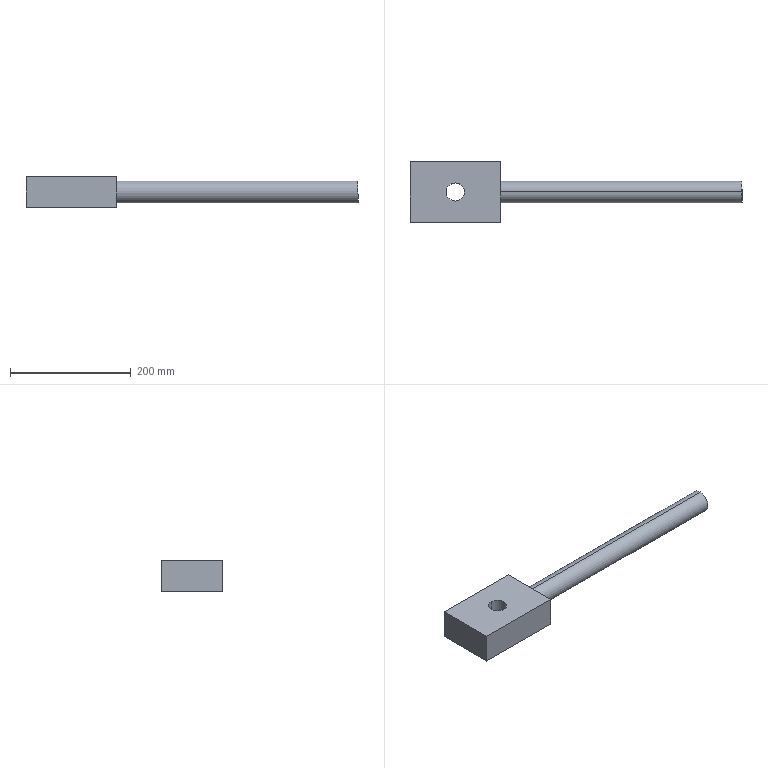Component | SolidWorks | 6TractionAxis-1 | 1 solid | 11 faces | box 550 x 100 x 50 mm | volume 1121807 mm3 | plane 7 | cylinder 4 | commonest cylinder face diameters 30 x2 36 x2
build123d program:
from build123d import *

# Parameters (mm, degrees)
SKETCH1_R           = 18
BOSS_EXTRUDE1_DEPTH = 400
SKETCH2_W           = 50
SKETCH2_H           = 100
BOSS_EXTRUDE2_DEPTH = 150
SKETCH3_R           = 15
CUT_EXTRUDE1_DEPTH  = 407.202


with BuildPart() as part:
    # Sketch1 → Boss-Extrude1 (new body)
    with BuildSketch(Plane.XY):
        Circle(SKETCH1_R)
    extrude(amount=BOSS_EXTRUDE1_DEPTH)

    # Sketch2 → Boss-Extrude2 (add)
    with BuildSketch(Plane(origin=(0, 0, 0), x_dir=(-1, 0, 0), z_dir=(0, 0, -1))):
        Rectangle(SKETCH2_W, SKETCH2_H)
    extrude(amount=BOSS_EXTRUDE2_DEPTH)

    # Sketch3 → Cut-Extrude1 (cut, through all)
    with BuildSketch(Plane.ZY.offset(25)):
        with Locations(Location((-75, 0, 0), (0, 0, 270))):
            Circle(SKETCH3_R)
    extrude(amount=-CUT_EXTRUDE1_DEPTH, mode=Mode.SUBTRACT)


solid = part.part

# Placed as in the assembly
solid = solid.moved(Location((-516.471, -3.79, 600), (0, 90, 0)))
STEP:
#1=CARTESIAN_POINT('',(-23.286,-0.7398,24.606));
#2=VERTEX_POINT('',#1);
#3=CARTESIAN_POINT('',(-23.286,0.4413,24.606));
#4=VERTEX_POINT('',#3);
#5=CARTESIAN_POINT('',(-23.286,-0.1492,24.606));
#6=DIRECTION('',(0.,-0.,-1.));
#7=DIRECTION('',(-0.,1.,0.));
#8=AXIS2_PLACEMENT_3D('',#5,#6,#7);
#9=CIRCLE('',#8,0.5906);
#10=EDGE_CURVE('',#2,#4,#9,.T.);
#11=ORIENTED_EDGE('',*,*,#10,.F.);
#12=CARTESIAN_POINT('',(-23.286,-0.7398,22.638));
#13=VERTEX_POINT('',#12);
#14=CARTESIAN_POINT('',(-23.286,-0.7398,24.606));
#15=DIRECTION('',(0.,-0.,-1.));
#16=VECTOR('',#15,39.37);
#17=LINE('',#14,#16);
#18=EDGE_CURVE('',#2,#13,#17,.T.);
#19=ORIENTED_EDGE('',*,*,#18,.T.);
#20=CARTESIAN_POINT('',(-23.286,0.4413,22.638));
#21=VERTEX_POINT('',#20);
#22=CARTESIAN_POINT('',(-23.286,-0.1492,22.638));
#23=DIRECTION('',(0.,-0.,-1.));
#24=DIRECTION('',(-0.,1.,0.));
#25=AXIS2_PLACEMENT_3D('',#22,#23,#24);
#26=CIRCLE('',#25,0.5906);
#27=EDGE_CURVE('',#13,#21,#26,.T.);
#28=ORIENTED_EDGE('',*,*,#27,.T.);
#29=CARTESIAN_POINT('',(-23.286,0.4413,24.606));
#30=DIRECTION('',(0.,-0.,-1.));
#31=VECTOR('',#30,39.37);
#32=LINE('',#29,#31);
#33=EDGE_CURVE('',#4,#21,#32,.T.);
#34=ORIENTED_EDGE('',*,*,#33,.F.);
#35=EDGE_LOOP('',(#11,#19,#28,#34));
#36=FACE_OUTER_BOUND('',#35,.T.);
#37=CARTESIAN_POINT('',(-23.286,-0.1492,24.606));
#38=DIRECTION('',(0.,-0.,-1.));
#39=DIRECTION('',(-0.,1.,0.));
#40=AXIS2_PLACEMENT_3D('',#37,#38,#39);
#41=CYLINDRICAL_SURFACE('',#40,0.5906);
#42=ADVANCED_FACE('',(#36),#41,.F.);
#43=CARTESIAN_POINT('',(-4.585,-0.1492,24.331));
#44=VERTEX_POINT('',#43);
#45=CARTESIAN_POINT('',(-4.585,-0.1492,22.913));
#46=VERTEX_POINT('',#45);
#47=CARTESIAN_POINT('',(-4.585,-0.1492,23.622));
#48=DIRECTION('',(1.,0.,0.));
#49=DIRECTION('',(-0.,0.,1.));
#50=AXIS2_PLACEMENT_3D('',#47,#48,#49);
#51=CIRCLE('',#50,0.7087);
#52=EDGE_CURVE('',#44,#46,#51,.T.);
#53=ORIENTED_EDGE('',*,*,#52,.F.);
#54=CARTESIAN_POINT('',(-20.333,-0.1492,24.331));
#55=VERTEX_POINT('',#54);
#56=CARTESIAN_POINT('',(-4.585,-0.1492,24.331));
#57=DIRECTION('',(-1.,-0.,-0.));
#58=VECTOR('',#57,39.37);
#59=LINE('',#56,#58);
#60=EDGE_CURVE('',#44,#55,#59,.T.);
#61=ORIENTED_EDGE('',*,*,#60,.T.);
#62=CARTESIAN_POINT('',(-20.333,-0.1492,22.913));
#63=VERTEX_POINT('',#62);
#64=CARTESIAN_POINT('',(-20.333,-0.1492,23.622));
#65=DIRECTION('',(1.,0.,0.));
#66=DIRECTION('',(-0.,0.,1.));
#67=AXIS2_PLACEMENT_3D('',#64,#65,#66);
#68=CIRCLE('',#67,0.7087);
#69=EDGE_CURVE('',#55,#63,#68,.T.);
#70=ORIENTED_EDGE('',*,*,#69,.T.);
#71=CARTESIAN_POINT('',(-4.585,-0.1492,22.913));
#72=DIRECTION('',(-1.,-0.,-0.));
#73=VECTOR('',#72,39.37);
#74=LINE('',#71,#73);
#75=EDGE_CURVE('',#46,#63,#74,.T.);
#76=ORIENTED_EDGE('',*,*,#75,.F.);
#77=EDGE_LOOP('',(#53,#61,#70,#76));
#78=FACE_OUTER_BOUND('',#77,.T.);
#79=CARTESIAN_POINT('',(-4.585,-0.1492,23.622));
#80=DIRECTION('',(-1.,-0.,-0.));
#81=DIRECTION('',(0.,0.,-1.));
#82=AXIS2_PLACEMENT_3D('',#79,#80,#81);
#83=CYLINDRICAL_SURFACE('',#82,0.7087);
#84=ADVANCED_FACE('',(#78),#83,.T.);
#85=ORIENTED_EDGE('',*,*,#60,.F.);
#86=CARTESIAN_POINT('',(-4.585,-0.1492,23.622));
#87=DIRECTION('',(1.,0.,0.));
#88=DIRECTION('',(-0.,0.,1.));
#89=AXIS2_PLACEMENT_3D('',#86,#87,#88);
#90=CIRCLE('',#89,0.7087);
#91=EDGE_CURVE('',#46,#44,#90,.T.);
#92=ORIENTED_EDGE('',*,*,#91,.F.);
#93=ORIENTED_EDGE('',*,*,#75,.T.);
#94=CARTESIAN_POINT('',(-20.333,-0.1492,23.622));
#95=DIRECTION('',(1.,0.,0.));
#96=DIRECTION('',(-0.,0.,1.));
#97=AXIS2_PLACEMENT_3D('',#94,#95,#96);
#98=CIRCLE('',#97,0.7087);
#99=EDGE_CURVE('',#63,#55,#98,.T.);
#100=ORIENTED_EDGE('',*,*,#99,.T.);
#101=EDGE_LOOP('',(#85,#92,#93,#100));
#102=FACE_OUTER_BOUND('',#101,.T.);
#103=CARTESIAN_POINT('',(-4.585,-0.1492,23.622));
#104=DIRECTION('',(-1.,-0.,-0.));
#105=DIRECTION('',(0.,0.,-1.));
#106=AXIS2_PLACEMENT_3D('',#103,#104,#105);
#107=CYLINDRICAL_SURFACE('',#106,0.7087);
#108=ADVANCED_FACE('',(#102),#107,.T.);
#109=ORIENTED_EDGE('',*,*,#91,.T.);
#110=ORIENTED_EDGE('',*,*,#52,.T.);
#111=EDGE_LOOP('',(#109,#110));
#112=FACE_OUTER_BOUND('',#111,.T.);
#113=CARTESIAN_POINT('',(-4.585,-0.1492,23.622));
#114=DIRECTION('',(1.,0.,0.));
#115=DIRECTION('',(-0.,-0.,1.));
#116=AXIS2_PLACEMENT_3D('',#113,#114,#115);
#117=PLANE('',#116);
#118=ADVANCED_FACE('',(#112),#117,.T.);
#119=CARTESIAN_POINT('',(-23.286,-0.1492,22.638));
#120=DIRECTION('',(0.,-0.,-1.));
#121=DIRECTION('',(-0.,1.,0.));
#122=AXIS2_PLACEMENT_3D('',#119,#120,#121);
#123=CIRCLE('',#122,0.5906);
#124=EDGE_CURVE('',#21,#13,#123,.T.);
#125=ORIENTED_EDGE('',*,*,#124,.F.);
#126=ORIENTED_EDGE('',*,*,#27,.F.);
#127=EDGE_LOOP('',(#125,#126));
#128=FACE_BOUND('',#127,.T.);
#129=CARTESIAN_POINT('',(-20.333,1.819,22.638));
#130=VERTEX_POINT('',#129);
#131=CARTESIAN_POINT('',(-20.333,-2.118,22.638));
#132=VERTEX_POINT('',#131);
#133=CARTESIAN_POINT('',(-20.333,-2.118,22.638));
#134=DIRECTION('',(0.,-1.,0.));
#135=VECTOR('',#134,39.37);
#136=LINE('',#133,#135);
#137=EDGE_CURVE('',#130,#132,#136,.T.);
#138=ORIENTED_EDGE('',*,*,#137,.T.);
#139=CARTESIAN_POINT('',(-26.239,-2.118,22.638));
#140=VERTEX_POINT('',#139);
#141=CARTESIAN_POINT('',(-26.239,-2.118,22.638));
#142=DIRECTION('',(1.,0.,0.));
#143=VECTOR('',#142,39.37);
#144=LINE('',#141,#143);
#145=EDGE_CURVE('',#140,#132,#144,.T.);
#146=ORIENTED_EDGE('',*,*,#145,.F.);
#147=CARTESIAN_POINT('',(-26.239,1.819,22.638));
#148=VERTEX_POINT('',#147);
#149=CARTESIAN_POINT('',(-26.239,-2.118,22.638));
#150=DIRECTION('',(0.,-1.,0.));
#151=VECTOR('',#150,39.37);
#152=LINE('',#149,#151);
#153=EDGE_CURVE('',#148,#140,#152,.T.);
#154=ORIENTED_EDGE('',*,*,#153,.F.);
#155=CARTESIAN_POINT('',(-26.239,1.819,22.638));
#156=DIRECTION('',(1.,0.,0.));
#157=VECTOR('',#156,39.37);
#158=LINE('',#155,#157);
#159=EDGE_CURVE('',#148,#130,#158,.T.);
#160=ORIENTED_EDGE('',*,*,#159,.T.);
#161=EDGE_LOOP('',(#138,#146,#154,#160));
#162=FACE_OUTER_BOUND('',#161,.T.);
#163=CARTESIAN_POINT('',(-26.239,-2.118,22.638));
#164=DIRECTION('',(-0.,0.,1.));
#165=DIRECTION('',(0.,-1.,0.));
#166=AXIS2_PLACEMENT_3D('',#163,#164,#165);
#167=PLANE('',#166);
#168=ADVANCED_FACE('',(#128,#162),#167,.F.);
#169=CARTESIAN_POINT('',(-20.333,-2.118,24.606));
#170=VERTEX_POINT('',#169);
#171=CARTESIAN_POINT('',(-20.333,-2.118,24.606));
#172=DIRECTION('',(-0.,-0.,1.));
#173=VECTOR('',#172,39.37);
#174=LINE('',#171,#173);
#175=EDGE_CURVE('',#132,#170,#174,.T.);
#176=ORIENTED_EDGE('',*,*,#175,.T.);
#177=CARTESIAN_POINT('',(-26.239,-2.118,24.606));
#178=VERTEX_POINT('',#177);
#179=CARTESIAN_POINT('',(-26.239,-2.118,24.606));
#180=DIRECTION('',(1.,0.,0.));
#181=VECTOR('',#180,39.37);
#182=LINE('',#179,#181);
#183=EDGE_CURVE('',#178,#170,#182,.T.);
#184=ORIENTED_EDGE('',*,*,#183,.F.);
#185=CARTESIAN_POINT('',(-26.239,-2.118,24.606));
#186=DIRECTION('',(-0.,-0.,1.));
#187=VECTOR('',#186,39.37);
#188=LINE('',#185,#187);
#189=EDGE_CURVE('',#140,#178,#188,.T.);
#190=ORIENTED_EDGE('',*,*,#189,.F.);
#191=ORIENTED_EDGE('',*,*,#145,.T.);
#192=EDGE_LOOP('',(#176,#184,#190,#191));
#193=FACE_OUTER_BOUND('',#192,.T.);
#194=CARTESIAN_POINT('',(-26.239,-2.118,24.606));
#195=DIRECTION('',(-0.,1.,-0.));
#196=DIRECTION('',(-1.,-0.,-0.));
#197=AXIS2_PLACEMENT_3D('',#194,#195,#196);
#198=PLANE('',#197);
#199=ADVANCED_FACE('',(#193),#198,.F.);
#200=CARTESIAN_POINT('',(-23.286,-0.1492,24.606));
#201=DIRECTION('',(0.,-0.,-1.));
#202=DIRECTION('',(-0.,1.,0.));
#203=AXIS2_PLACEMENT_3D('',#200,#201,#202);
#204=CIRCLE('',#203,0.5906);
#205=EDGE_CURVE('',#4,#2,#204,.T.);
#206=ORIENTED_EDGE('',*,*,#205,.T.);
#207=ORIENTED_EDGE('',*,*,#10,.T.);
#208=EDGE_LOOP('',(#206,#207));
#209=FACE_BOUND('',#208,.T.);
#210=CARTESIAN_POINT('',(-20.333,1.819,24.606));
#211=VERTEX_POINT('',#210);
#212=CARTESIAN_POINT('',(-20.333,-2.118,24.606));
#213=DIRECTION('',(-0.,1.,-0.));
#214=VECTOR('',#213,39.37);
#215=LINE('',#212,#214);
#216=EDGE_CURVE('',#170,#211,#215,.T.);
#217=ORIENTED_EDGE('',*,*,#216,.T.);
#218=CARTESIAN_POINT('',(-26.239,1.819,24.606));
#219=VERTEX_POINT('',#218);
#220=CARTESIAN_POINT('',(-26.239,1.819,24.606));
#221=DIRECTION('',(1.,0.,0.));
#222=VECTOR('',#221,39.37);
#223=LINE('',#220,#222);
#224=EDGE_CURVE('',#219,#211,#223,.T.);
#225=ORIENTED_EDGE('',*,*,#224,.F.);
#226=CARTESIAN_POINT('',(-26.239,-2.118,24.606));
#227=DIRECTION('',(-0.,1.,-0.));
#228=VECTOR('',#227,39.37);
#229=LINE('',#226,#228);
#230=EDGE_CURVE('',#178,#219,#229,.T.);
#231=ORIENTED_EDGE('',*,*,#230,.F.);
#232=ORIENTED_EDGE('',*,*,#183,.T.);
#233=EDGE_LOOP('',(#217,#225,#231,#232));
#234=FACE_OUTER_BOUND('',#233,.T.);
#235=CARTESIAN_POINT('',(-26.239,-2.118,24.606));
#236=DIRECTION('',(0.,-0.,-1.));
#237=DIRECTION('',(-0.,1.,-0.));
#238=AXIS2_PLACEMENT_3D('',#235,#236,#237);
#239=PLANE('',#238);
#240=ADVANCED_FACE('',(#209,#234),#239,.F.);
#241=CARTESIAN_POINT('',(-20.333,1.819,24.606));
#242=DIRECTION('',(0.,0.,-1.));
#243=VECTOR('',#242,39.37);
#244=LINE('',#241,#243);
#245=EDGE_CURVE('',#211,#130,#244,.T.);
#246=ORIENTED_EDGE('',*,*,#245,.T.);
#247=ORIENTED_EDGE('',*,*,#159,.F.);
#248=CARTESIAN_POINT('',(-26.239,1.819,24.606));
#249=DIRECTION('',(0.,0.,-1.));
#250=VECTOR('',#249,39.37);
#251=LINE('',#248,#250);
#252=EDGE_CURVE('',#219,#148,#251,.T.);
#253=ORIENTED_EDGE('',*,*,#252,.F.);
#254=ORIENTED_EDGE('',*,*,#224,.T.);
#255=EDGE_LOOP('',(#246,#247,#253,#254));
#256=FACE_OUTER_BOUND('',#255,.T.);
#257=CARTESIAN_POINT('',(-26.239,1.819,24.606));
#258=DIRECTION('',(0.,-1.,0.));
#259=DIRECTION('',(1.,0.,0.));
#260=AXIS2_PLACEMENT_3D('',#257,#258,#259);
#261=PLANE('',#260);
#262=ADVANCED_FACE('',(#256),#261,.F.);
#263=ORIENTED_EDGE('',*,*,#153,.T.);
#264=ORIENTED_EDGE('',*,*,#189,.T.);
#265=ORIENTED_EDGE('',*,*,#230,.T.);
#266=ORIENTED_EDGE('',*,*,#252,.T.);
#267=EDGE_LOOP('',(#263,#264,#265,#266));
#268=FACE_OUTER_BOUND('',#267,.T.);
#269=CARTESIAN_POINT('',(-26.239,-0.1492,23.622));
#270=DIRECTION('',(-1.,-0.,-0.));
#271=DIRECTION('',(0.,0.,-1.));
#272=AXIS2_PLACEMENT_3D('',#269,#270,#271);
#273=PLANE('',#272);
#274=ADVANCED_FACE('',(#268),#273,.T.);
#275=ORIENTED_EDGE('',*,*,#99,.F.);
#276=ORIENTED_EDGE('',*,*,#69,.F.);
#277=EDGE_LOOP('',(#275,#276));
#278=FACE_BOUND('',#277,.T.);
#279=ORIENTED_EDGE('',*,*,#137,.F.);
#280=ORIENTED_EDGE('',*,*,#245,.F.);
#281=ORIENTED_EDGE('',*,*,#216,.F.);
#282=ORIENTED_EDGE('',*,*,#175,.F.);
#283=EDGE_LOOP('',(#279,#280,#281,#282));
#284=FACE_OUTER_BOUND('',#283,.T.);
#285=CARTESIAN_POINT('',(-20.333,-0.1492,23.622));
#286=DIRECTION('',(-1.,-0.,-0.));
#287=DIRECTION('',(0.,0.,-1.));
#288=AXIS2_PLACEMENT_3D('',#285,#286,#287);
#289=PLANE('',#288);
#290=ADVANCED_FACE('',(#278,#284),#289,.F.);
#291=ORIENTED_EDGE('',*,*,#18,.F.);
#292=ORIENTED_EDGE('',*,*,#205,.F.);
#293=ORIENTED_EDGE('',*,*,#33,.T.);
#294=ORIENTED_EDGE('',*,*,#124,.T.);
#295=EDGE_LOOP('',(#291,#292,#293,#294));
#296=FACE_OUTER_BOUND('',#295,.T.);
#297=CARTESIAN_POINT('',(-23.286,-0.1492,24.606));
#298=DIRECTION('',(0.,-0.,-1.));
#299=DIRECTION('',(-0.,1.,0.));
#300=AXIS2_PLACEMENT_3D('',#297,#298,#299);
#301=CYLINDRICAL_SURFACE('',#300,0.5906);
#302=ADVANCED_FACE('',(#296),#301,.F.);
#303=CLOSED_SHELL('',(#42,#84,#108,#118,#168,#199,#240,#262,#274,#290,#302));
#304=MANIFOLD_SOLID_BREP('',#303);
#305=CARTESIAN_POINT('',(0.,0.,0.));
#306=DIRECTION('',(0.,0.,1.));
#307=DIRECTION('',(1.,0.,0.));
#308=AXIS2_PLACEMENT_3D('',#305,#306,#307);
#309=(LENGTH_UNIT()NAMED_UNIT(*)SI_UNIT($,.METRE.));
#310=LENGTH_MEASURE_WITH_UNIT(LENGTH_MEASURE(0.0254),#309);
#311=DIMENSIONAL_EXPONENTS(1.,0.,0.,0.,0.,0.,0.);
#312=(CONVERSION_BASED_UNIT('',#310)LENGTH_UNIT()NAMED_UNIT(#311));
#313=UNCERTAINTY_MEASURE_WITH_UNIT(LENGTH_MEASURE(0.00001),#312,'','');
#314=(NAMED_UNIT(*)PLANE_ANGLE_UNIT()SI_UNIT($,.RADIAN.));
#315=(NAMED_UNIT(*)SI_UNIT($,.STERADIAN.)SOLID_ANGLE_UNIT());
#316=(GEOMETRIC_REPRESENTATION_CONTEXT(3)GLOBAL_UNCERTAINTY_ASSIGNED_CONTEXT((#313))GLOBAL_UNIT_ASSIGNED_CONTEXT((#312,#314,#315))REPRESENTATION_CONTEXT('',''));
#317=ADVANCED_BREP_SHAPE_REPRESENTATION('',(#304,#308),#316);
#318=COLOUR_RGB('',0.7922,0.8196,0.9333);
#319=FILL_AREA_STYLE_COLOUR('',#318);
#320=FILL_AREA_STYLE('',(#319));
#321=SURFACE_STYLE_FILL_AREA(#320);
#322=SURFACE_SIDE_STYLE('',(#321));
#323=SURFACE_STYLE_USAGE(.BOTH.,#322);
#324=PRESENTATION_STYLE_ASSIGNMENT((#323));
#325=STYLED_ITEM('',(#324),#304);
#326=(LENGTH_UNIT()NAMED_UNIT(*)SI_UNIT($,.METRE.));
#327=LENGTH_MEASURE_WITH_UNIT(LENGTH_MEASURE(0.0254),#326);
#328=DIMENSIONAL_EXPONENTS(1.,0.,0.,0.,0.,0.,0.);
#329=(CONVERSION_BASED_UNIT('',#327)LENGTH_UNIT()NAMED_UNIT(#328));
#330=UNCERTAINTY_MEASURE_WITH_UNIT(LENGTH_MEASURE(0.00001),#329,'','');
#331=(NAMED_UNIT(*)PLANE_ANGLE_UNIT()SI_UNIT($,.RADIAN.));
#332=(NAMED_UNIT(*)SI_UNIT($,.STERADIAN.)SOLID_ANGLE_UNIT());
#333=(GEOMETRIC_REPRESENTATION_CONTEXT(3)GLOBAL_UNCERTAINTY_ASSIGNED_CONTEXT((#330))GLOBAL_UNIT_ASSIGNED_CONTEXT((#329,#331,#332))REPRESENTATION_CONTEXT('',''));
#334=MECHANICAL_DESIGN_GEOMETRIC_PRESENTATION_REPRESENTATION('',(#325),#333);
#335=PRESENTATION_LAYER_ASSIGNMENT('','',(#325));